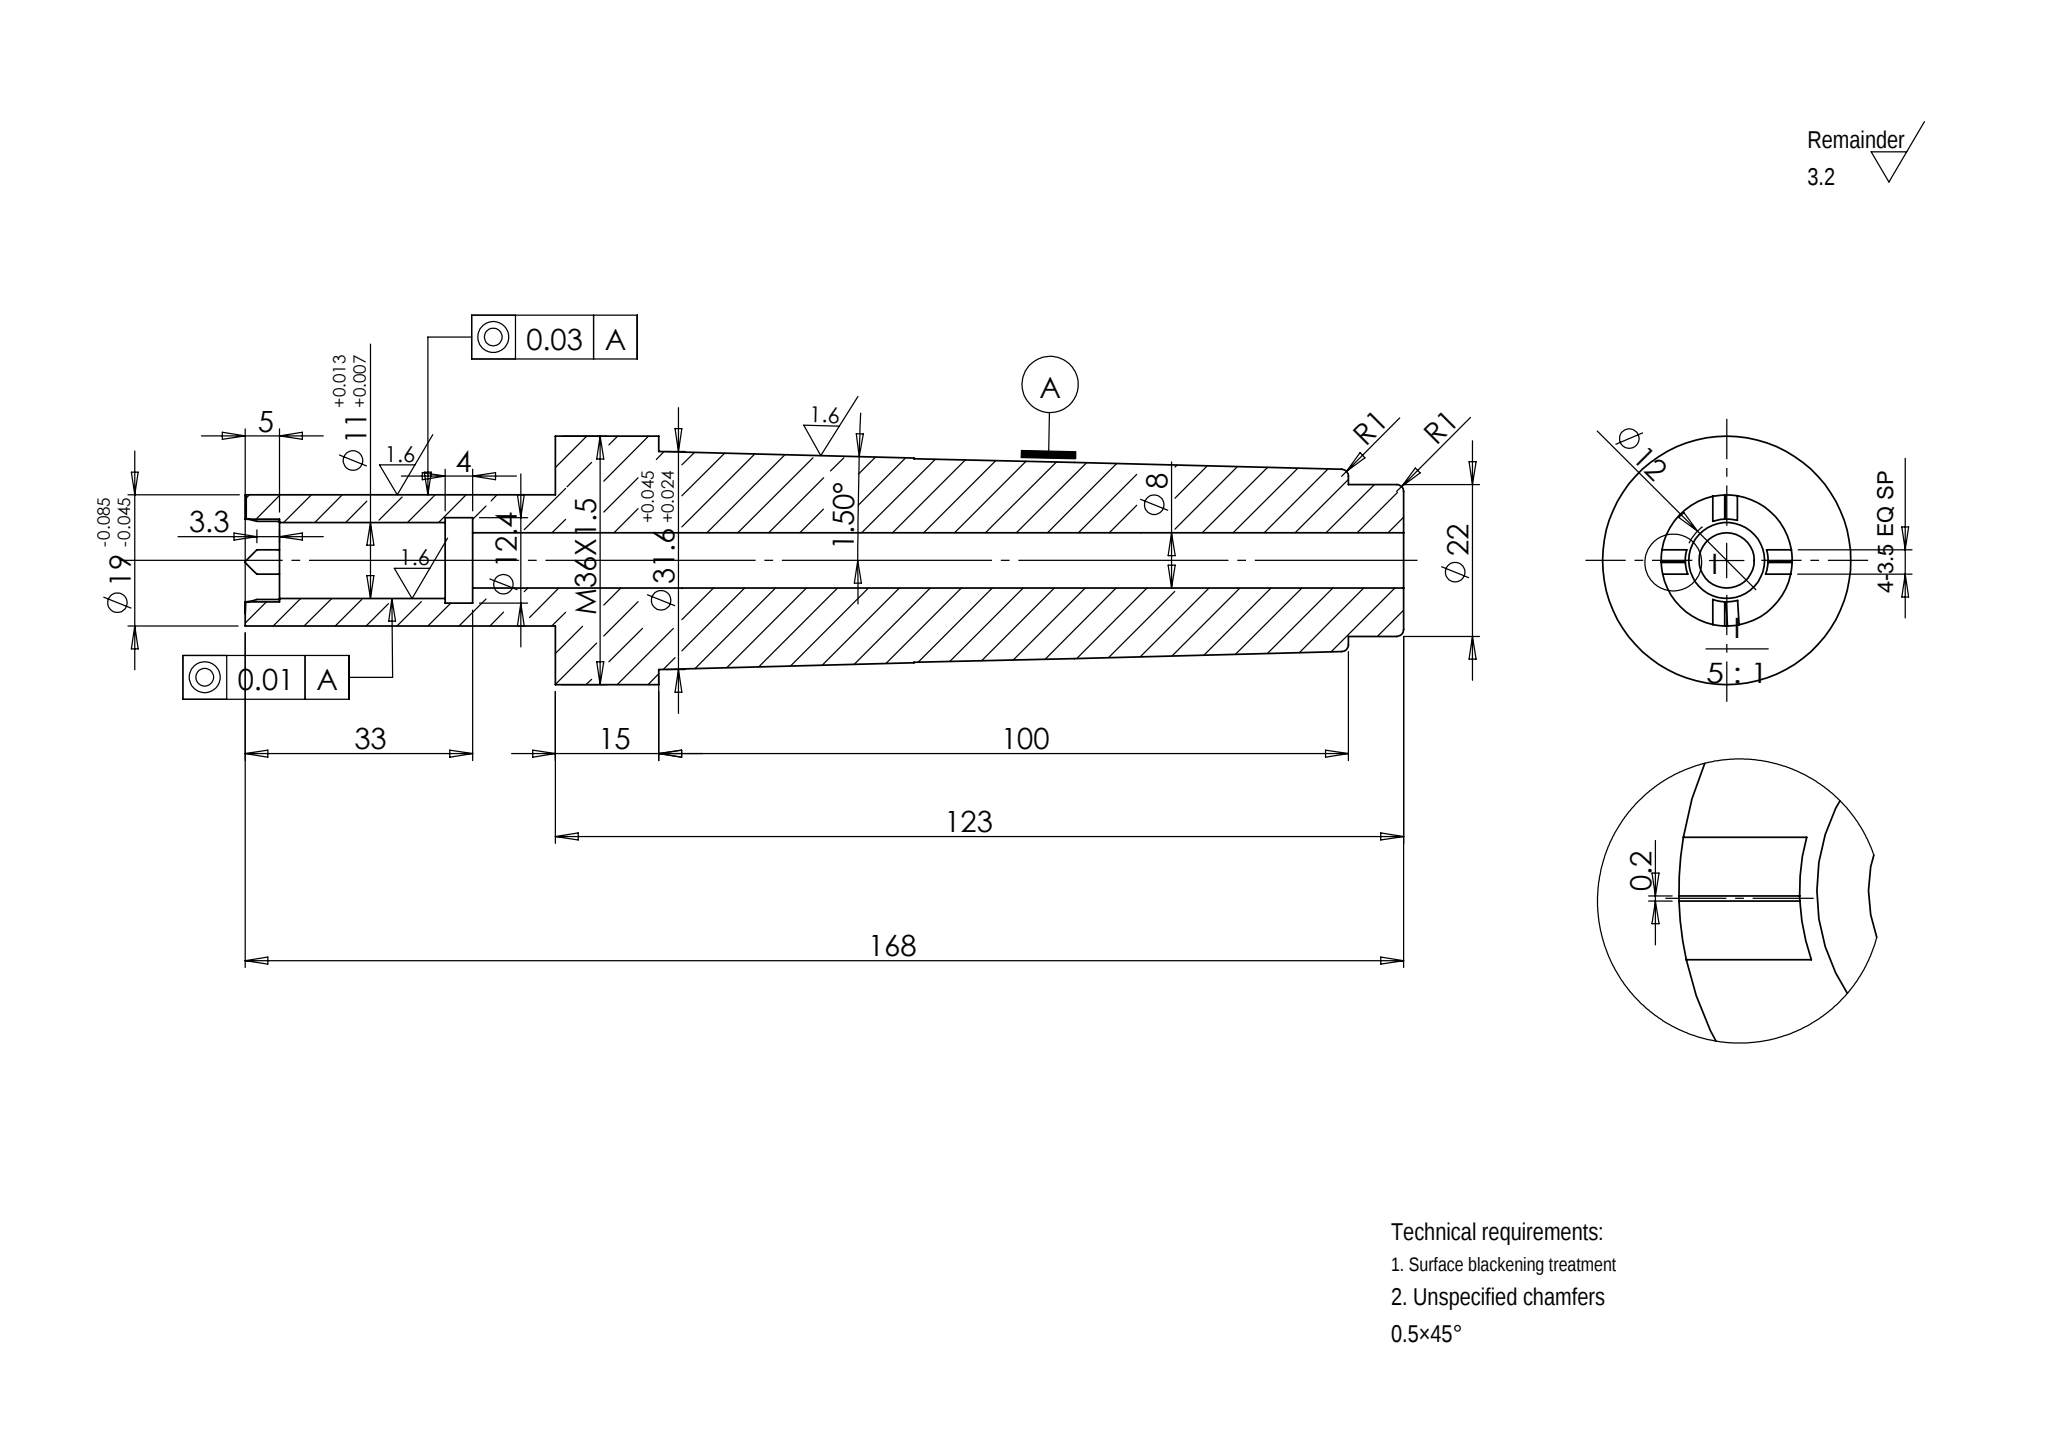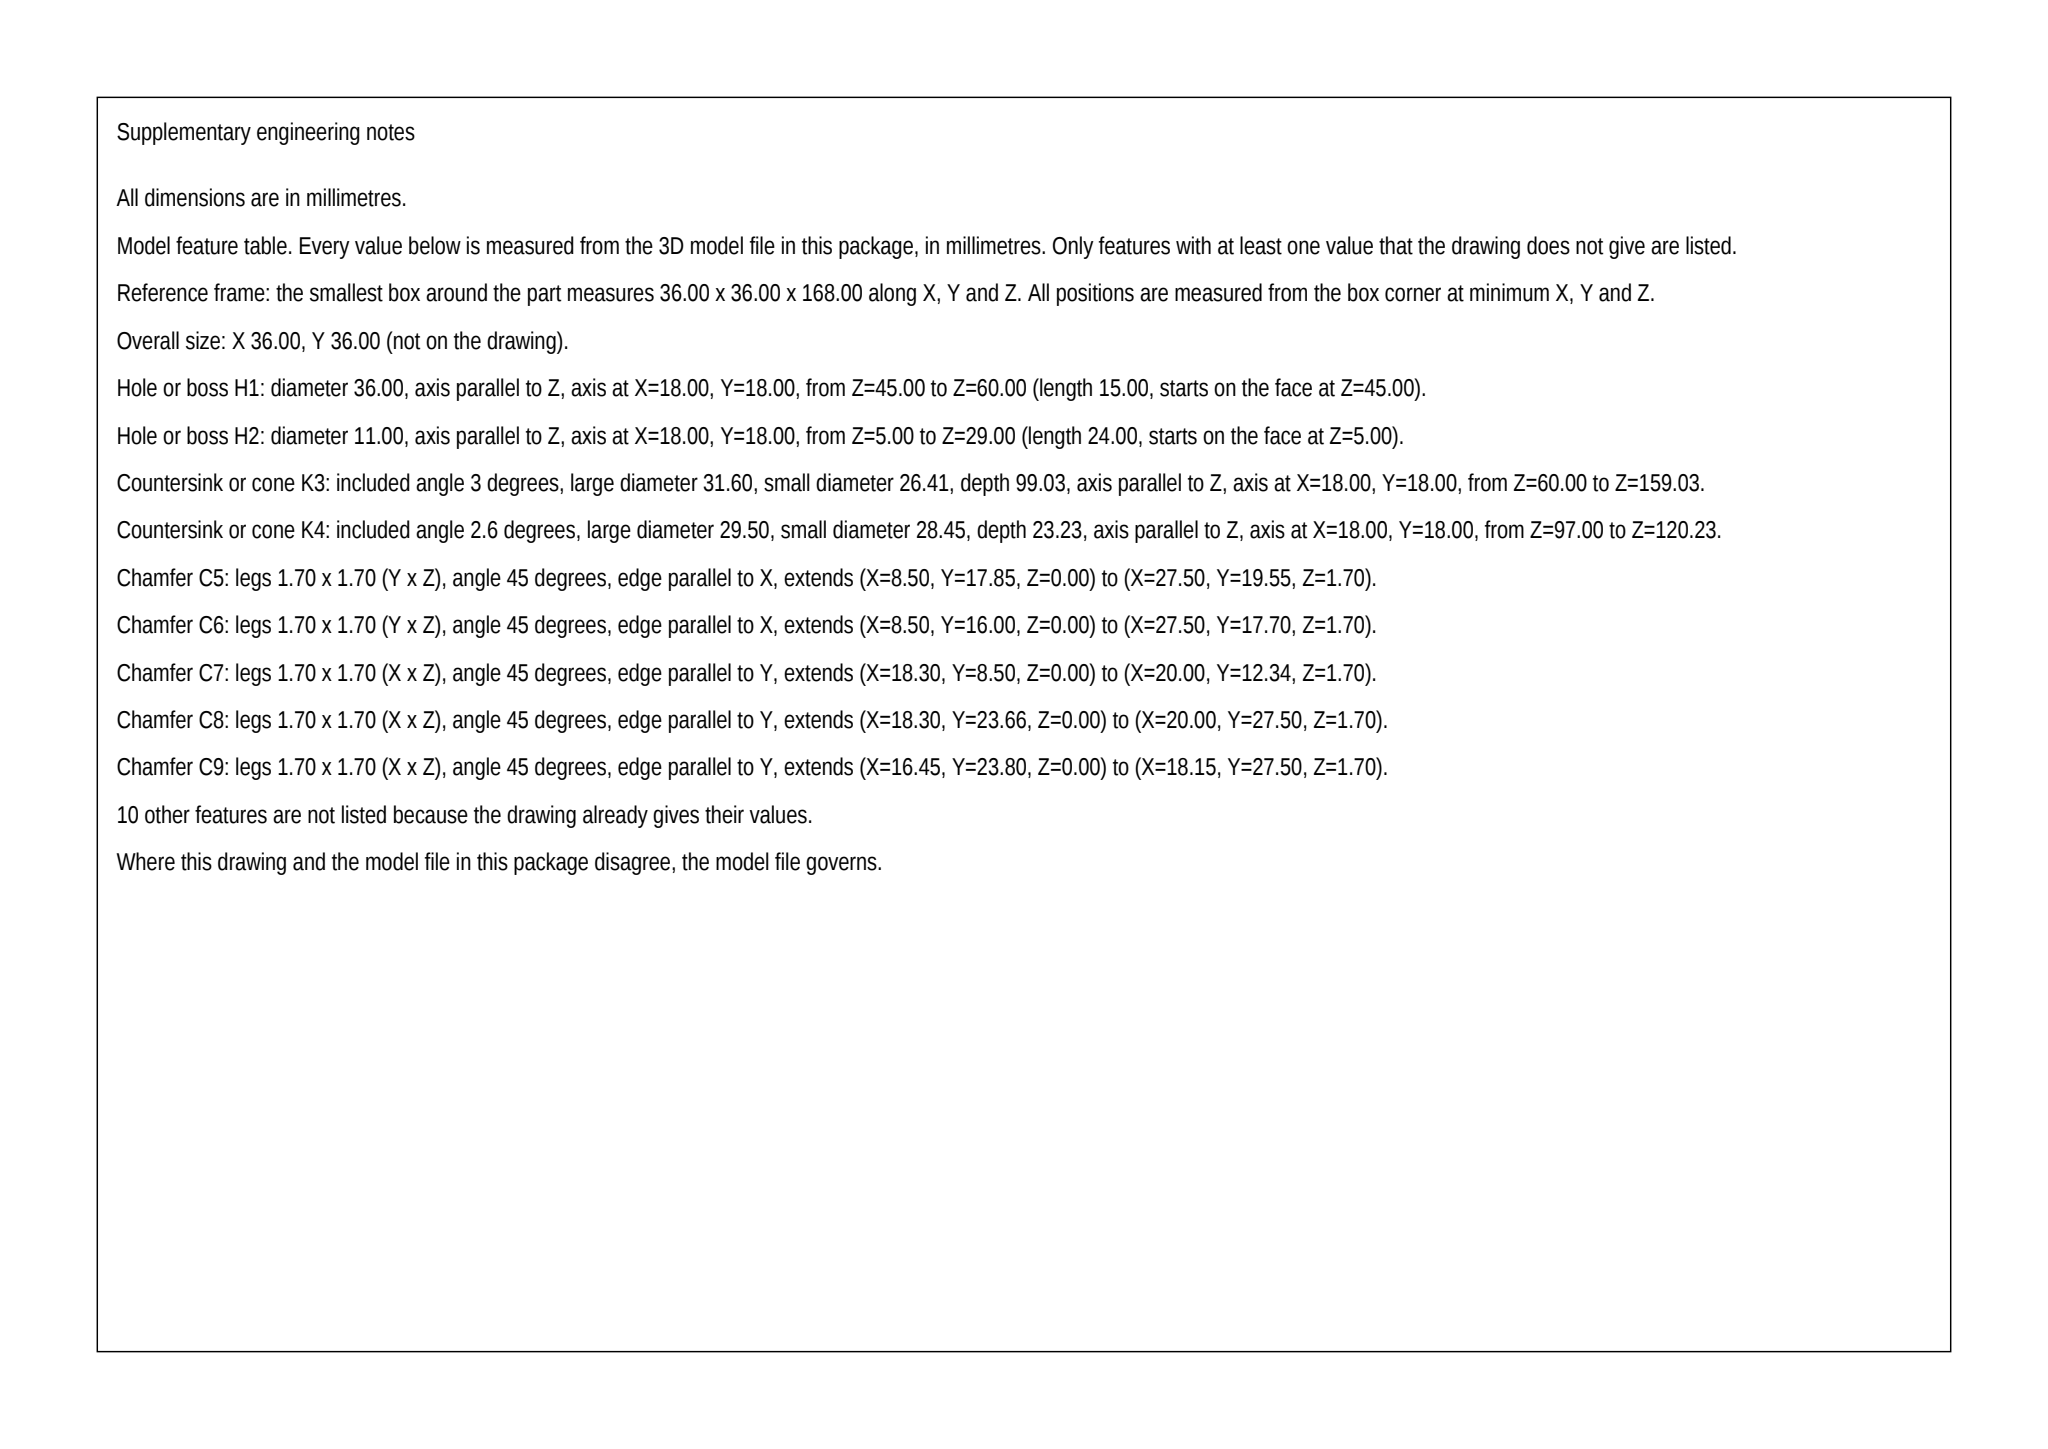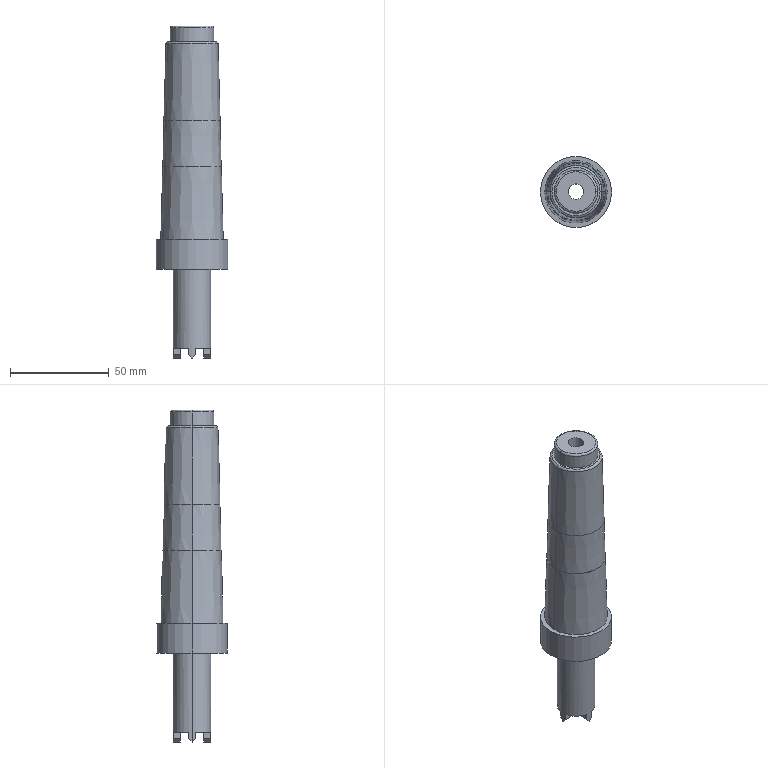Part | SolidWorks | mm | 1 solid | 55 faces | box 36 x 36 x 168 mm | volume 86343 mm3 | plane 28 | cylinder 17 | cone 6 | torus 4 | commonest cylinder face diameters 12 x5 12.4 x2 8 x2 22 x2 36 x2 19 x2 11 x2